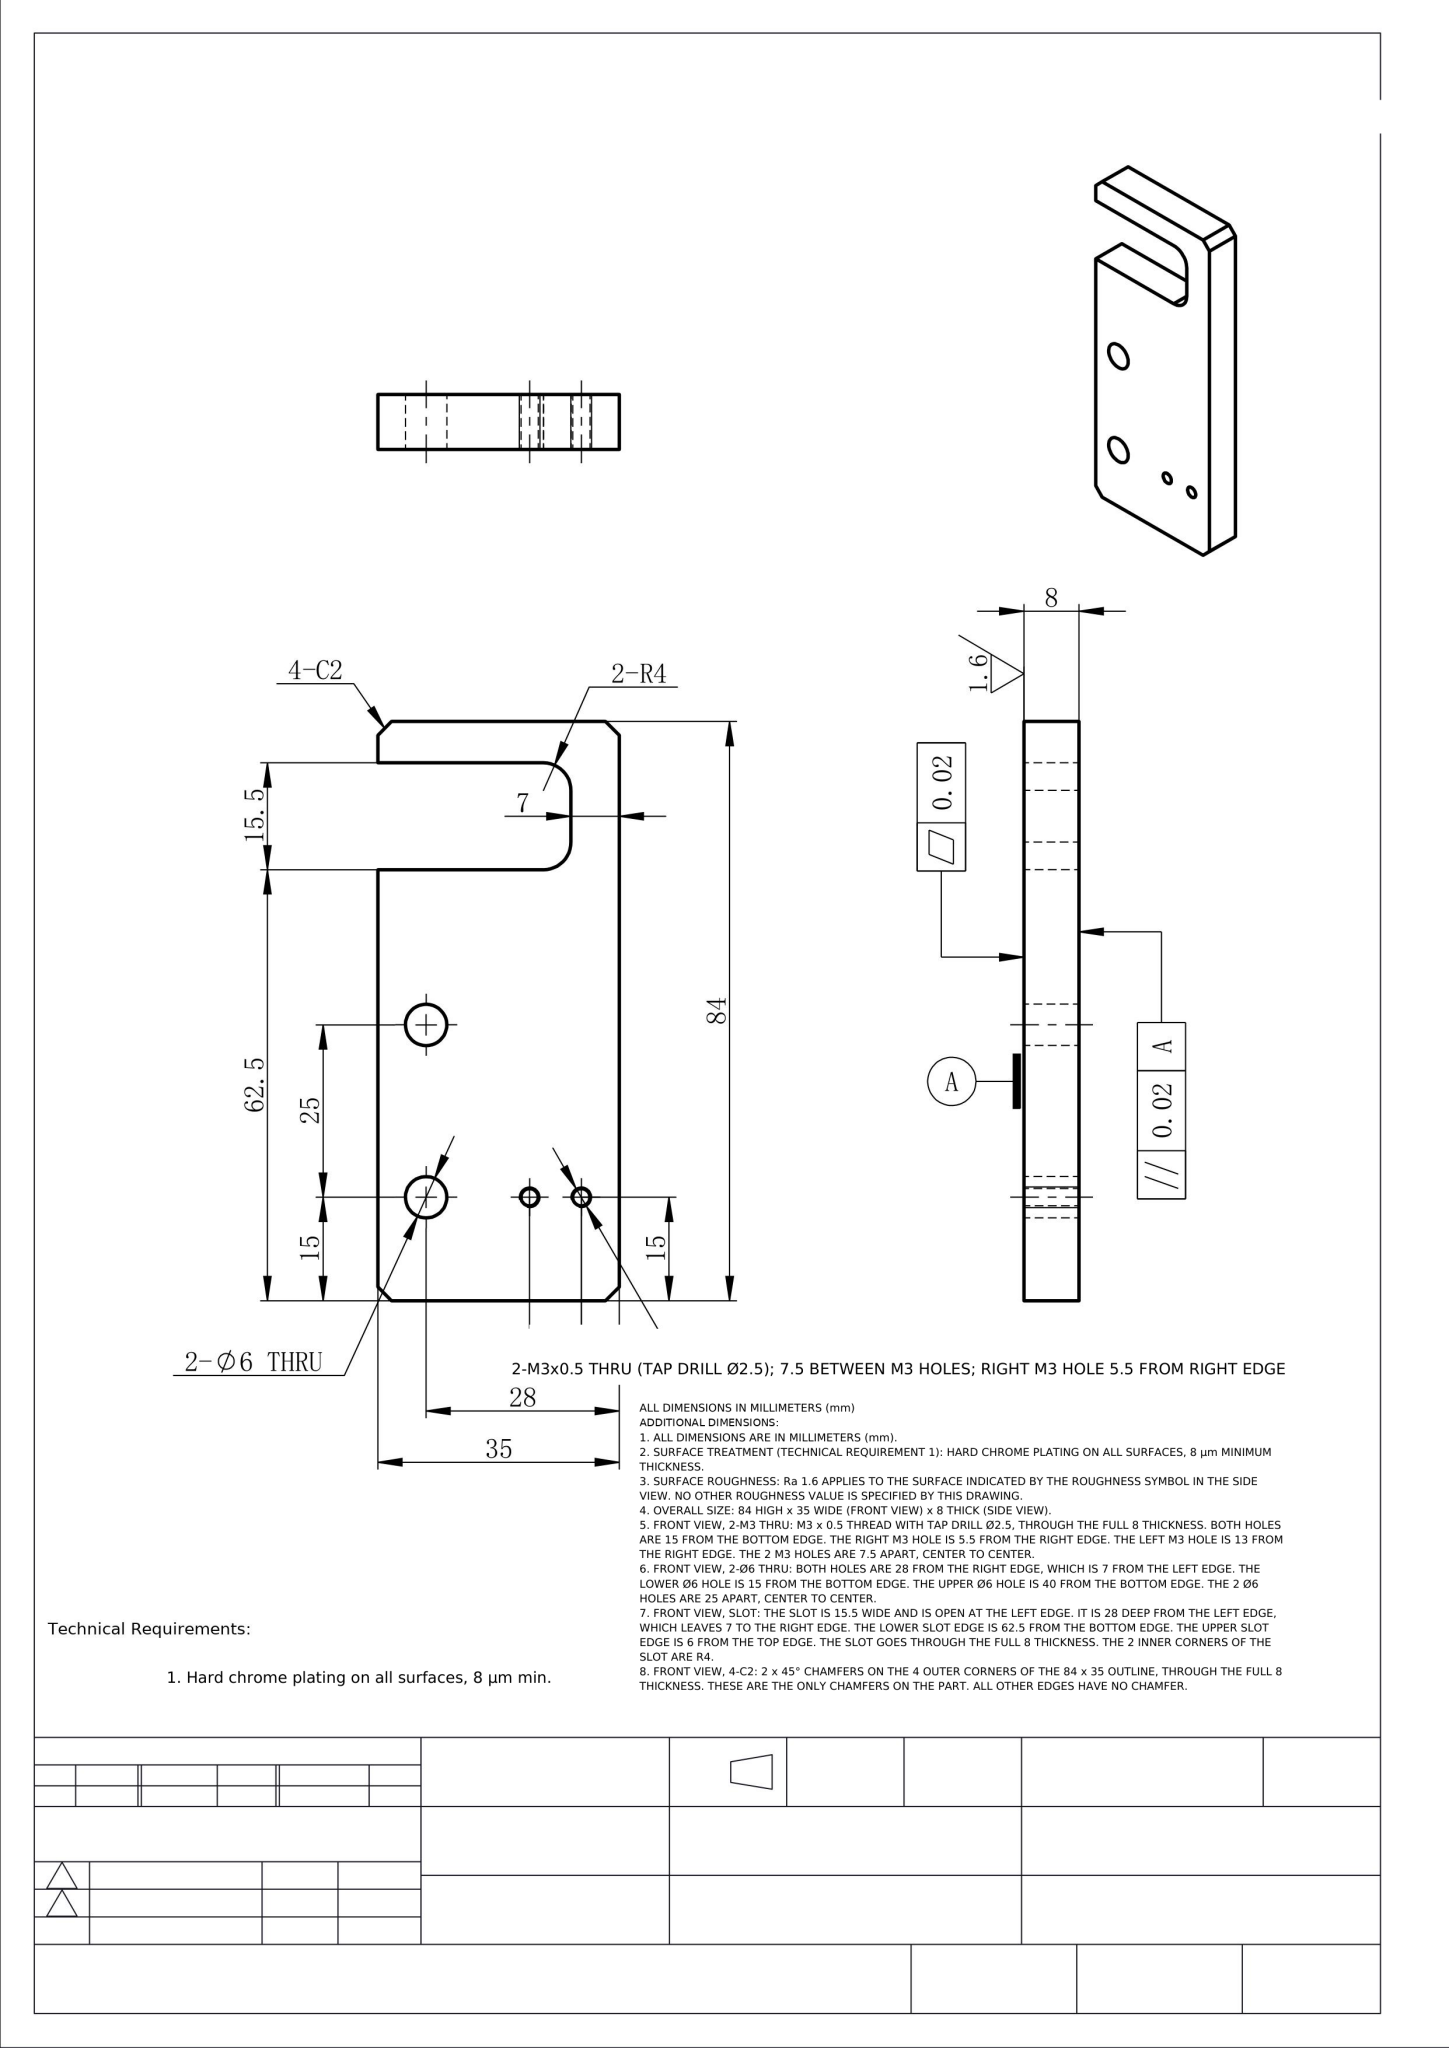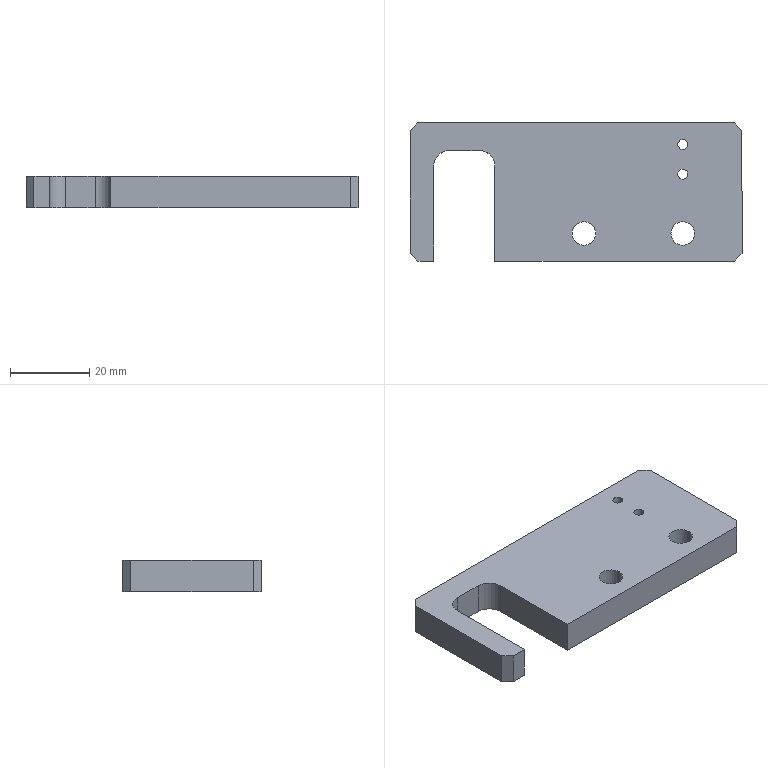Part | NX | mm | 1 solid | 24 faces | box 84 x 35 x 8 mm | volume 19508 mm3 | plane 14 | cylinder 10 | commonest cylinder face diameters 2.5 x4 6 x4 8 x2
STEP:
#1=COLOUR_RGB('',0.7961,0.8235,0.9373);
#2=FILL_AREA_STYLE_COLOUR('',#1);
#3=FILL_AREA_STYLE('',(#2));
#4=SURFACE_STYLE_FILL_AREA(#3);
#5=SURFACE_SIDE_STYLE('',(#4));
#6=SURFACE_STYLE_USAGE(.BOTH.,#5);
#7=PRESENTATION_STYLE_ASSIGNMENT((#6));
#8=CARTESIAN_POINT('',(-16.25,-5.5,-4.));
#9=VERTEX_POINT('',#8);
#10=CARTESIAN_POINT('',(-16.25,-5.5,4.));
#11=VERTEX_POINT('',#10);
#12=CARTESIAN_POINT('',(-16.25,-5.5,4.));
#13=DIRECTION('',(0.,0.,1.));
#14=VECTOR('',#13,1000.);
#15=LINE('',#12,#14);
#16=EDGE_CURVE('',#9,#11,#15,.T.);
#17=ORIENTED_EDGE('',*,*,#16,.F.);
#18=CARTESIAN_POINT('',(-13.75,-5.5,-4.));
#19=VERTEX_POINT('',#18);
#20=CARTESIAN_POINT('',(-15.,-5.5,-4.));
#21=DIRECTION('',(0.,0.,1.));
#22=DIRECTION('',(1.,0.,0.));
#23=AXIS2_PLACEMENT_3D('',#20,#21,#22);
#24=CIRCLE('',#23,1.25);
#25=EDGE_CURVE('',#19,#9,#24,.T.);
#26=ORIENTED_EDGE('',*,*,#25,.F.);
#27=CARTESIAN_POINT('',(-13.75,-5.5,4.));
#28=VERTEX_POINT('',#27);
#29=CARTESIAN_POINT('',(-13.75,-5.5,4.));
#30=DIRECTION('',(0.,0.,1.));
#31=VECTOR('',#30,1000.);
#32=LINE('',#29,#31);
#33=EDGE_CURVE('',#19,#28,#32,.T.);
#34=ORIENTED_EDGE('',*,*,#33,.T.);
#35=CARTESIAN_POINT('',(-15.,-5.5,4.));
#36=DIRECTION('',(0.,0.,1.));
#37=DIRECTION('',(1.,0.,0.));
#38=AXIS2_PLACEMENT_3D('',#35,#36,#37);
#39=CIRCLE('',#38,1.25);
#40=EDGE_CURVE('',#28,#11,#39,.T.);
#41=ORIENTED_EDGE('',*,*,#40,.T.);
#42=EDGE_LOOP('',(#17,#26,#34,#41));
#43=FACE_OUTER_BOUND('',#42,.T.);
#44=CARTESIAN_POINT('',(-15.,-5.5,4.));
#45=DIRECTION('',(0.,0.,1.));
#46=DIRECTION('',(1.,0.,0.));
#47=AXIS2_PLACEMENT_3D('',#44,#45,#46);
#48=CYLINDRICAL_SURFACE('',#47,1.25);
#49=ADVANCED_FACE('',(#43),#48,.F.);
#50=STYLED_ITEM('',(#7),#49);
#51=(LENGTH_UNIT()NAMED_UNIT(*)SI_UNIT(.MILLI.,.METRE.));
#52=UNCERTAINTY_MEASURE_WITH_UNIT(LENGTH_MEASURE(0.00001),#51,'','');
#53=(NAMED_UNIT(*)PLANE_ANGLE_UNIT()SI_UNIT($,.RADIAN.));
#54=(NAMED_UNIT(*)SI_UNIT($,.STERADIAN.)SOLID_ANGLE_UNIT());
#55=(GEOMETRIC_REPRESENTATION_CONTEXT(3)GLOBAL_UNCERTAINTY_ASSIGNED_CONTEXT((#52))GLOBAL_UNIT_ASSIGNED_CONTEXT((#51,#53,#54))REPRESENTATION_CONTEXT('',''));
#56=MECHANICAL_DESIGN_GEOMETRIC_PRESENTATION_REPRESENTATION('',(#50),#55);
#57=COLOUR_RGB('',0.7961,0.8235,0.9373);
#58=FILL_AREA_STYLE_COLOUR('',#57);
#59=FILL_AREA_STYLE('',(#58));
#60=SURFACE_STYLE_FILL_AREA(#59);
#61=SURFACE_SIDE_STYLE('',(#60));
#62=SURFACE_STYLE_USAGE(.BOTH.,#61);
#63=PRESENTATION_STYLE_ASSIGNMENT((#62));
#64=CARTESIAN_POINT('',(-15.,-5.5,-4.));
#65=DIRECTION('',(0.,0.,1.));
#66=DIRECTION('',(1.,0.,0.));
#67=AXIS2_PLACEMENT_3D('',#64,#65,#66);
#68=CIRCLE('',#67,1.25);
#69=EDGE_CURVE('',#9,#19,#68,.T.);
#70=ORIENTED_EDGE('',*,*,#69,.F.);
#71=ORIENTED_EDGE('',*,*,#16,.T.);
#72=CARTESIAN_POINT('',(-15.,-5.5,4.));
#73=DIRECTION('',(0.,0.,1.));
#74=DIRECTION('',(1.,0.,0.));
#75=AXIS2_PLACEMENT_3D('',#72,#73,#74);
#76=CIRCLE('',#75,1.25);
#77=EDGE_CURVE('',#11,#28,#76,.T.);
#78=ORIENTED_EDGE('',*,*,#77,.T.);
#79=ORIENTED_EDGE('',*,*,#33,.F.);
#80=EDGE_LOOP('',(#70,#71,#78,#79));
#81=FACE_OUTER_BOUND('',#80,.T.);
#82=CARTESIAN_POINT('',(-15.,-5.5,4.));
#83=DIRECTION('',(0.,0.,1.));
#84=DIRECTION('',(1.,0.,0.));
#85=AXIS2_PLACEMENT_3D('',#82,#83,#84);
#86=CYLINDRICAL_SURFACE('',#85,1.25);
#87=ADVANCED_FACE('',(#81),#86,.F.);
#88=CARTESIAN_POINT('',(-16.25,-13.,-4.));
#89=VERTEX_POINT('',#88);
#90=CARTESIAN_POINT('',(-13.75,-13.,-4.));
#91=VERTEX_POINT('',#90);
#92=CARTESIAN_POINT('',(-15.,-13.,-4.));
#93=DIRECTION('',(0.,0.,1.));
#94=DIRECTION('',(1.,0.,0.));
#95=AXIS2_PLACEMENT_3D('',#92,#93,#94);
#96=CIRCLE('',#95,1.25);
#97=EDGE_CURVE('',#89,#91,#96,.T.);
#98=ORIENTED_EDGE('',*,*,#97,.F.);
#99=CARTESIAN_POINT('',(-16.25,-13.,4.));
#100=VERTEX_POINT('',#99);
#101=CARTESIAN_POINT('',(-16.25,-13.,4.));
#102=DIRECTION('',(0.,0.,1.));
#103=VECTOR('',#102,1000.);
#104=LINE('',#101,#103);
#105=EDGE_CURVE('',#89,#100,#104,.T.);
#106=ORIENTED_EDGE('',*,*,#105,.T.);
#107=CARTESIAN_POINT('',(-13.75,-13.,4.));
#108=VERTEX_POINT('',#107);
#109=CARTESIAN_POINT('',(-15.,-13.,4.));
#110=DIRECTION('',(0.,0.,1.));
#111=DIRECTION('',(1.,0.,0.));
#112=AXIS2_PLACEMENT_3D('',#109,#110,#111);
#113=CIRCLE('',#112,1.25);
#114=EDGE_CURVE('',#100,#108,#113,.T.);
#115=ORIENTED_EDGE('',*,*,#114,.T.);
#116=CARTESIAN_POINT('',(-13.75,-13.,4.));
#117=DIRECTION('',(0.,0.,1.));
#118=VECTOR('',#117,1000.);
#119=LINE('',#116,#118);
#120=EDGE_CURVE('',#91,#108,#119,.T.);
#121=ORIENTED_EDGE('',*,*,#120,.F.);
#122=EDGE_LOOP('',(#98,#106,#115,#121));
#123=FACE_OUTER_BOUND('',#122,.T.);
#124=CARTESIAN_POINT('',(-15.,-13.,4.));
#125=DIRECTION('',(0.,0.,1.));
#126=DIRECTION('',(1.,0.,0.));
#127=AXIS2_PLACEMENT_3D('',#124,#125,#126);
#128=CYLINDRICAL_SURFACE('',#127,1.25);
#129=ADVANCED_FACE('',(#123),#128,.F.);
#130=CARTESIAN_POINT('',(-18.,-28.,-4.));
#131=VERTEX_POINT('',#130);
#132=CARTESIAN_POINT('',(-12.,-28.,-4.));
#133=VERTEX_POINT('',#132);
#134=CARTESIAN_POINT('',(-15.,-28.,-4.));
#135=DIRECTION('',(0.,0.,1.));
#136=DIRECTION('',(1.,0.,0.));
#137=AXIS2_PLACEMENT_3D('',#134,#135,#136);
#138=CIRCLE('',#137,3.);
#139=EDGE_CURVE('',#131,#133,#138,.T.);
#140=ORIENTED_EDGE('',*,*,#139,.F.);
#141=CARTESIAN_POINT('',(-18.,-28.,4.));
#142=VERTEX_POINT('',#141);
#143=CARTESIAN_POINT('',(-18.,-28.,-4.));
#144=DIRECTION('',(0.,0.,1.));
#145=VECTOR('',#144,1000.);
#146=LINE('',#143,#145);
#147=EDGE_CURVE('',#131,#142,#146,.T.);
#148=ORIENTED_EDGE('',*,*,#147,.T.);
#149=CARTESIAN_POINT('',(-12.,-28.,4.));
#150=VERTEX_POINT('',#149);
#151=CARTESIAN_POINT('',(-15.,-28.,4.));
#152=DIRECTION('',(0.,0.,1.));
#153=DIRECTION('',(1.,0.,0.));
#154=AXIS2_PLACEMENT_3D('',#151,#152,#153);
#155=CIRCLE('',#154,3.);
#156=EDGE_CURVE('',#142,#150,#155,.T.);
#157=ORIENTED_EDGE('',*,*,#156,.T.);
#158=CARTESIAN_POINT('',(-12.,-28.,-4.));
#159=DIRECTION('',(0.,0.,1.));
#160=VECTOR('',#159,1000.);
#161=LINE('',#158,#160);
#162=EDGE_CURVE('',#133,#150,#161,.T.);
#163=ORIENTED_EDGE('',*,*,#162,.F.);
#164=EDGE_LOOP('',(#140,#148,#157,#163));
#165=FACE_OUTER_BOUND('',#164,.T.);
#166=CARTESIAN_POINT('',(-15.,-28.,-4.));
#167=DIRECTION('',(0.,0.,1.));
#168=DIRECTION('',(1.,0.,0.));
#169=AXIS2_PLACEMENT_3D('',#166,#167,#168);
#170=CYLINDRICAL_SURFACE('',#169,3.);
#171=ADVANCED_FACE('',(#165),#170,.F.);
#172=CARTESIAN_POINT('',(-43.,-28.,-4.));
#173=VERTEX_POINT('',#172);
#174=CARTESIAN_POINT('',(-37.,-28.,-4.));
#175=VERTEX_POINT('',#174);
#176=CARTESIAN_POINT('',(-40.,-28.,-4.));
#177=DIRECTION('',(0.,0.,1.));
#178=DIRECTION('',(1.,0.,0.));
#179=AXIS2_PLACEMENT_3D('',#176,#177,#178);
#180=CIRCLE('',#179,3.);
#181=EDGE_CURVE('',#173,#175,#180,.T.);
#182=ORIENTED_EDGE('',*,*,#181,.F.);
#183=CARTESIAN_POINT('',(-43.,-28.,4.));
#184=VERTEX_POINT('',#183);
#185=CARTESIAN_POINT('',(-43.,-28.,-4.));
#186=DIRECTION('',(0.,0.,1.));
#187=VECTOR('',#186,1000.);
#188=LINE('',#185,#187);
#189=EDGE_CURVE('',#173,#184,#188,.T.);
#190=ORIENTED_EDGE('',*,*,#189,.T.);
#191=CARTESIAN_POINT('',(-37.,-28.,4.));
#192=VERTEX_POINT('',#191);
#193=CARTESIAN_POINT('',(-40.,-28.,4.));
#194=DIRECTION('',(0.,0.,1.));
#195=DIRECTION('',(1.,0.,0.));
#196=AXIS2_PLACEMENT_3D('',#193,#194,#195);
#197=CIRCLE('',#196,3.);
#198=EDGE_CURVE('',#184,#192,#197,.T.);
#199=ORIENTED_EDGE('',*,*,#198,.T.);
#200=CARTESIAN_POINT('',(-37.,-28.,-4.));
#201=DIRECTION('',(0.,0.,1.));
#202=VECTOR('',#201,1000.);
#203=LINE('',#200,#202);
#204=EDGE_CURVE('',#175,#192,#203,.T.);
#205=ORIENTED_EDGE('',*,*,#204,.F.);
#206=EDGE_LOOP('',(#182,#190,#199,#205));
#207=FACE_OUTER_BOUND('',#206,.T.);
#208=CARTESIAN_POINT('',(-40.,-28.,-4.));
#209=DIRECTION('',(0.,0.,1.));
#210=DIRECTION('',(1.,0.,0.));
#211=AXIS2_PLACEMENT_3D('',#208,#209,#210);
#212=CYLINDRICAL_SURFACE('',#211,3.);
#213=ADVANCED_FACE('',(#207),#212,.F.);
#214=CARTESIAN_POINT('',(0.,-33.,4.));
#215=VERTEX_POINT('',#214);
#216=CARTESIAN_POINT('',(0.,-2.,4.));
#217=VERTEX_POINT('',#216);
#218=CARTESIAN_POINT('',(0.,0.,4.));
#219=DIRECTION('',(-0.,1.,0.));
#220=VECTOR('',#219,1000.);
#221=LINE('',#218,#220);
#222=EDGE_CURVE('',#215,#217,#221,.T.);
#223=ORIENTED_EDGE('',*,*,#222,.F.);
#224=CARTESIAN_POINT('',(0.,-33.,-4.));
#225=VERTEX_POINT('',#224);
#226=CARTESIAN_POINT('',(0.,-33.,4.));
#227=DIRECTION('',(0.,0.,-1.));
#228=VECTOR('',#227,1000.);
#229=LINE('',#226,#228);
#230=EDGE_CURVE('',#215,#225,#229,.T.);
#231=ORIENTED_EDGE('',*,*,#230,.T.);
#232=CARTESIAN_POINT('',(0.,-2.,-4.));
#233=VERTEX_POINT('',#232);
#234=CARTESIAN_POINT('',(0.,0.,-4.));
#235=DIRECTION('',(-0.,1.,0.));
#236=VECTOR('',#235,1000.);
#237=LINE('',#234,#236);
#238=EDGE_CURVE('',#225,#233,#237,.T.);
#239=ORIENTED_EDGE('',*,*,#238,.T.);
#240=CARTESIAN_POINT('',(0.,-2.,4.));
#241=DIRECTION('',(0.,0.,1.));
#242=VECTOR('',#241,1000.);
#243=LINE('',#240,#242);
#244=EDGE_CURVE('',#233,#217,#243,.T.);
#245=ORIENTED_EDGE('',*,*,#244,.T.);
#246=EDGE_LOOP('',(#223,#231,#239,#245));
#247=FACE_OUTER_BOUND('',#246,.T.);
#248=CARTESIAN_POINT('',(0.,0.,4.));
#249=DIRECTION('',(-1.,-0.,0.));
#250=DIRECTION('',(0.,-1.,0.));
#251=AXIS2_PLACEMENT_3D('',#248,#249,#250);
#252=PLANE('',#251);
#253=ADVANCED_FACE('',(#247),#252,.F.);
#254=CARTESIAN_POINT('',(-2.,-0.,4.));
#255=VERTEX_POINT('',#254);
#256=CARTESIAN_POINT('',(-82.,-0.,4.));
#257=VERTEX_POINT('',#256);
#258=CARTESIAN_POINT('',(0.,0.,4.));
#259=DIRECTION('',(-1.,-0.,0.));
#260=VECTOR('',#259,1000.);
#261=LINE('',#258,#260);
#262=EDGE_CURVE('',#255,#257,#261,.T.);
#263=ORIENTED_EDGE('',*,*,#262,.F.);
#264=CARTESIAN_POINT('',(-2.,0.,-4.));
#265=VERTEX_POINT('',#264);
#266=CARTESIAN_POINT('',(-2.,-0.,4.));
#267=DIRECTION('',(0.,0.,-1.));
#268=VECTOR('',#267,1000.);
#269=LINE('',#266,#268);
#270=EDGE_CURVE('',#255,#265,#269,.T.);
#271=ORIENTED_EDGE('',*,*,#270,.T.);
#272=CARTESIAN_POINT('',(-82.,-0.,-4.));
#273=VERTEX_POINT('',#272);
#274=CARTESIAN_POINT('',(0.,0.,-4.));
#275=DIRECTION('',(-1.,-0.,0.));
#276=VECTOR('',#275,1000.);
#277=LINE('',#274,#276);
#278=EDGE_CURVE('',#265,#273,#277,.T.);
#279=ORIENTED_EDGE('',*,*,#278,.T.);
#280=CARTESIAN_POINT('',(-82.,-0.,4.));
#281=DIRECTION('',(0.,0.,1.));
#282=VECTOR('',#281,1000.);
#283=LINE('',#280,#282);
#284=EDGE_CURVE('',#273,#257,#283,.T.);
#285=ORIENTED_EDGE('',*,*,#284,.T.);
#286=EDGE_LOOP('',(#263,#271,#279,#285));
#287=FACE_OUTER_BOUND('',#286,.T.);
#288=CARTESIAN_POINT('',(0.,0.,4.));
#289=DIRECTION('',(0.,-1.,0.));
#290=DIRECTION('',(1.,0.,0.));
#291=AXIS2_PLACEMENT_3D('',#288,#289,#290);
#292=PLANE('',#291);
#293=ADVANCED_FACE('',(#287),#292,.F.);
#294=CARTESIAN_POINT('',(-84.,-2.,-4.));
#295=VERTEX_POINT('',#294);
#296=CARTESIAN_POINT('',(-84.,-33.,-4.));
#297=VERTEX_POINT('',#296);
#298=CARTESIAN_POINT('',(-84.,-35.,-4.));
#299=DIRECTION('',(0.,-1.,0.));
#300=VECTOR('',#299,1000.);
#301=LINE('',#298,#300);
#302=EDGE_CURVE('',#295,#297,#301,.T.);
#303=ORIENTED_EDGE('',*,*,#302,.T.);
#304=CARTESIAN_POINT('',(-84.,-33.,4.));
#305=VERTEX_POINT('',#304);
#306=CARTESIAN_POINT('',(-84.,-33.,4.));
#307=DIRECTION('',(0.,0.,1.));
#308=VECTOR('',#307,1000.);
#309=LINE('',#306,#308);
#310=EDGE_CURVE('',#297,#305,#309,.T.);
#311=ORIENTED_EDGE('',*,*,#310,.T.);
#312=CARTESIAN_POINT('',(-84.,-2.,4.));
#313=VERTEX_POINT('',#312);
#314=CARTESIAN_POINT('',(-84.,-35.,4.));
#315=DIRECTION('',(0.,-1.,0.));
#316=VECTOR('',#315,1000.);
#317=LINE('',#314,#316);
#318=EDGE_CURVE('',#313,#305,#317,.T.);
#319=ORIENTED_EDGE('',*,*,#318,.F.);
#320=CARTESIAN_POINT('',(-84.,-2.,4.));
#321=DIRECTION('',(0.,0.,-1.));
#322=VECTOR('',#321,1000.);
#323=LINE('',#320,#322);
#324=EDGE_CURVE('',#313,#295,#323,.T.);
#325=ORIENTED_EDGE('',*,*,#324,.T.);
#326=EDGE_LOOP('',(#303,#311,#319,#325));
#327=FACE_OUTER_BOUND('',#326,.T.);
#328=CARTESIAN_POINT('',(-84.,-35.,4.));
#329=DIRECTION('',(1.,0.,0.));
#330=DIRECTION('',(0.,0.,-1.));
#331=AXIS2_PLACEMENT_3D('',#328,#329,#330);
#332=PLANE('',#331);
#333=ADVANCED_FACE('',(#327),#332,.F.);
#334=CARTESIAN_POINT('',(-82.,-35.,4.));
#335=VERTEX_POINT('',#334);
#336=CARTESIAN_POINT('',(-78.,-35.,4.));
#337=VERTEX_POINT('',#336);
#338=CARTESIAN_POINT('',(-78.,-35.,4.));
#339=DIRECTION('',(1.,-0.,0.));
#340=VECTOR('',#339,1000.);
#341=LINE('',#338,#340);
#342=EDGE_CURVE('',#335,#337,#341,.T.);
#343=ORIENTED_EDGE('',*,*,#342,.F.);
#344=CARTESIAN_POINT('',(-82.,-35.,-4.));
#345=VERTEX_POINT('',#344);
#346=CARTESIAN_POINT('',(-82.,-35.,4.));
#347=DIRECTION('',(0.,0.,-1.));
#348=VECTOR('',#347,1000.);
#349=LINE('',#346,#348);
#350=EDGE_CURVE('',#335,#345,#349,.T.);
#351=ORIENTED_EDGE('',*,*,#350,.T.);
#352=CARTESIAN_POINT('',(-78.,-35.,-4.));
#353=VERTEX_POINT('',#352);
#354=CARTESIAN_POINT('',(-78.,-35.,-4.));
#355=DIRECTION('',(1.,-0.,0.));
#356=VECTOR('',#355,1000.);
#357=LINE('',#354,#356);
#358=EDGE_CURVE('',#345,#353,#357,.T.);
#359=ORIENTED_EDGE('',*,*,#358,.T.);
#360=CARTESIAN_POINT('',(-78.,-35.,4.));
#361=DIRECTION('',(0.,0.,-1.));
#362=VECTOR('',#361,1000.);
#363=LINE('',#360,#362);
#364=EDGE_CURVE('',#337,#353,#363,.T.);
#365=ORIENTED_EDGE('',*,*,#364,.F.);
#366=EDGE_LOOP('',(#343,#351,#359,#365));
#367=FACE_OUTER_BOUND('',#366,.T.);
#368=CARTESIAN_POINT('',(-78.,-35.,4.));
#369=DIRECTION('',(0.,1.,0.));
#370=DIRECTION('',(-1.,0.,0.));
#371=AXIS2_PLACEMENT_3D('',#368,#369,#370);
#372=PLANE('',#371);
#373=ADVANCED_FACE('',(#367),#372,.F.);
#374=CARTESIAN_POINT('',(-78.,-11.,-4.));
#375=VERTEX_POINT('',#374);
#376=CARTESIAN_POINT('',(-78.,-7.,-4.));
#377=DIRECTION('',(0.,1.,0.));
#378=VECTOR('',#377,1000.);
#379=LINE('',#376,#378);
#380=EDGE_CURVE('',#353,#375,#379,.T.);
#381=ORIENTED_EDGE('',*,*,#380,.T.);
#382=CARTESIAN_POINT('',(-78.,-11.,4.));
#383=VERTEX_POINT('',#382);
#384=CARTESIAN_POINT('',(-78.,-11.,4.));
#385=DIRECTION('',(0.,0.,1.));
#386=VECTOR('',#385,1000.);
#387=LINE('',#384,#386);
#388=EDGE_CURVE('',#375,#383,#387,.T.);
#389=ORIENTED_EDGE('',*,*,#388,.T.);
#390=CARTESIAN_POINT('',(-78.,-7.,4.));
#391=DIRECTION('',(0.,1.,0.));
#392=VECTOR('',#391,1000.);
#393=LINE('',#390,#392);
#394=EDGE_CURVE('',#337,#383,#393,.T.);
#395=ORIENTED_EDGE('',*,*,#394,.F.);
#396=ORIENTED_EDGE('',*,*,#364,.T.);
#397=EDGE_LOOP('',(#381,#389,#395,#396));
#398=FACE_OUTER_BOUND('',#397,.T.);
#399=CARTESIAN_POINT('',(-78.,-7.,4.));
#400=DIRECTION('',(-1.,0.,0.));
#401=DIRECTION('',(0.,0.,1.));
#402=AXIS2_PLACEMENT_3D('',#399,#400,#401);
#403=PLANE('',#402);
#404=ADVANCED_FACE('',(#398),#403,.F.);
#405=CARTESIAN_POINT('',(-74.,-7.,-4.));
#406=VERTEX_POINT('',#405);
#407=CARTESIAN_POINT('',(-66.5,-7.,-4.));
#408=VERTEX_POINT('',#407);
#409=CARTESIAN_POINT('',(-62.5,-7.,-4.));
#410=DIRECTION('',(1.,0.,0.));
#411=VECTOR('',#410,1000.);
#412=LINE('',#409,#411);
#413=EDGE_CURVE('',#406,#408,#412,.T.);
#414=ORIENTED_EDGE('',*,*,#413,.T.);
#415=CARTESIAN_POINT('',(-66.5,-7.,4.));
#416=VERTEX_POINT('',#415);
#417=CARTESIAN_POINT('',(-66.5,-7.,4.));
#418=DIRECTION('',(0.,0.,1.));
#419=VECTOR('',#418,1000.);
#420=LINE('',#417,#419);
#421=EDGE_CURVE('',#408,#416,#420,.T.);
#422=ORIENTED_EDGE('',*,*,#421,.T.);
#423=CARTESIAN_POINT('',(-74.,-7.,4.));
#424=VERTEX_POINT('',#423);
#425=CARTESIAN_POINT('',(-62.5,-7.,4.));
#426=DIRECTION('',(1.,0.,0.));
#427=VECTOR('',#426,1000.);
#428=LINE('',#425,#427);
#429=EDGE_CURVE('',#424,#416,#428,.T.);
#430=ORIENTED_EDGE('',*,*,#429,.F.);
#431=CARTESIAN_POINT('',(-74.,-7.,-4.));
#432=DIRECTION('',(0.,0.,-1.));
#433=VECTOR('',#432,1000.);
#434=LINE('',#431,#433);
#435=EDGE_CURVE('',#424,#406,#434,.T.);
#436=ORIENTED_EDGE('',*,*,#435,.T.);
#437=EDGE_LOOP('',(#414,#422,#430,#436));
#438=FACE_OUTER_BOUND('',#437,.T.);
#439=CARTESIAN_POINT('',(-62.5,-7.,4.));
#440=DIRECTION('',(-0.,1.,0.));
#441=DIRECTION('',(-1.,-0.,0.));
#442=AXIS2_PLACEMENT_3D('',#439,#440,#441);
#443=PLANE('',#442);
#444=ADVANCED_FACE('',(#438),#443,.F.);
#445=CARTESIAN_POINT('',(-62.5,-11.,4.));
#446=VERTEX_POINT('',#445);
#447=CARTESIAN_POINT('',(-62.5,-35.,4.));
#448=VERTEX_POINT('',#447);
#449=CARTESIAN_POINT('',(-62.5,-35.,4.));
#450=DIRECTION('',(0.,-1.,0.));
#451=VECTOR('',#450,1000.);
#452=LINE('',#449,#451);
#453=EDGE_CURVE('',#446,#448,#452,.T.);
#454=ORIENTED_EDGE('',*,*,#453,.F.);
#455=CARTESIAN_POINT('',(-62.5,-11.,-4.));
#456=VERTEX_POINT('',#455);
#457=CARTESIAN_POINT('',(-62.5,-11.,-4.));
#458=DIRECTION('',(0.,0.,-1.));
#459=VECTOR('',#458,1000.);
#460=LINE('',#457,#459);
#461=EDGE_CURVE('',#446,#456,#460,.T.);
#462=ORIENTED_EDGE('',*,*,#461,.T.);
#463=CARTESIAN_POINT('',(-62.5,-35.,-4.));
#464=VERTEX_POINT('',#463);
#465=CARTESIAN_POINT('',(-62.5,-35.,-4.));
#466=DIRECTION('',(0.,-1.,0.));
#467=VECTOR('',#466,1000.);
#468=LINE('',#465,#467);
#469=EDGE_CURVE('',#456,#464,#468,.T.);
#470=ORIENTED_EDGE('',*,*,#469,.T.);
#471=CARTESIAN_POINT('',(-62.5,-35.,4.));
#472=DIRECTION('',(0.,0.,-1.));
#473=VECTOR('',#472,1000.);
#474=LINE('',#471,#473);
#475=EDGE_CURVE('',#448,#464,#474,.T.);
#476=ORIENTED_EDGE('',*,*,#475,.F.);
#477=EDGE_LOOP('',(#454,#462,#470,#476));
#478=FACE_OUTER_BOUND('',#477,.T.);
#479=CARTESIAN_POINT('',(-62.5,-35.,4.));
#480=DIRECTION('',(1.,0.,0.));
#481=DIRECTION('',(0.,0.,-1.));
#482=AXIS2_PLACEMENT_3D('',#479,#480,#481);
#483=PLANE('',#482);
#484=ADVANCED_FACE('',(#478),#483,.F.);
#485=CARTESIAN_POINT('',(-2.,-35.,-4.));
#486=VERTEX_POINT('',#485);
#487=CARTESIAN_POINT('',(0.,-35.,-4.));
#488=DIRECTION('',(1.,0.,0.));
#489=VECTOR('',#488,1000.);
#490=LINE('',#487,#489);
#491=EDGE_CURVE('',#464,#486,#490,.T.);
#492=ORIENTED_EDGE('',*,*,#491,.T.);
#493=CARTESIAN_POINT('',(-2.,-35.,4.));
#494=VERTEX_POINT('',#493);
#495=CARTESIAN_POINT('',(-2.,-35.,4.));
#496=DIRECTION('',(0.,0.,1.));
#497=VECTOR('',#496,1000.);
#498=LINE('',#495,#497);
#499=EDGE_CURVE('',#486,#494,#498,.T.);
#500=ORIENTED_EDGE('',*,*,#499,.T.);
#501=CARTESIAN_POINT('',(0.,-35.,4.));
#502=DIRECTION('',(1.,0.,0.));
#503=VECTOR('',#502,1000.);
#504=LINE('',#501,#503);
#505=EDGE_CURVE('',#448,#494,#504,.T.);
#506=ORIENTED_EDGE('',*,*,#505,.F.);
#507=ORIENTED_EDGE('',*,*,#475,.T.);
#508=EDGE_LOOP('',(#492,#500,#506,#507));
#509=FACE_OUTER_BOUND('',#508,.T.);
#510=CARTESIAN_POINT('',(0.,-35.,4.));
#511=DIRECTION('',(-0.,1.,0.));
#512=DIRECTION('',(-1.,-0.,0.));
#513=AXIS2_PLACEMENT_3D('',#510,#511,#512);
#514=PLANE('',#513);
#515=ADVANCED_FACE('',(#509),#514,.F.);
#516=ORIENTED_EDGE('',*,*,#40,.F.);
#517=ORIENTED_EDGE('',*,*,#77,.F.);
#518=EDGE_LOOP('',(#516,#517));
#519=FACE_BOUND('',#518,.T.);
#520=CARTESIAN_POINT('',(-15.,-13.,4.));
#521=DIRECTION('',(0.,0.,1.));
#522=DIRECTION('',(1.,0.,0.));
#523=AXIS2_PLACEMENT_3D('',#520,#521,#522);
#524=CIRCLE('',#523,1.25);
#525=EDGE_CURVE('',#108,#100,#524,.T.);
#526=ORIENTED_EDGE('',*,*,#525,.F.);
#527=ORIENTED_EDGE('',*,*,#114,.F.);
#528=EDGE_LOOP('',(#526,#527));
#529=FACE_BOUND('',#528,.T.);
#530=CARTESIAN_POINT('',(-15.,-28.,4.));
#531=DIRECTION('',(0.,0.,1.));
#532=DIRECTION('',(1.,0.,0.));
#533=AXIS2_PLACEMENT_3D('',#530,#531,#532);
#534=CIRCLE('',#533,3.);
#535=EDGE_CURVE('',#150,#142,#534,.T.);
#536=ORIENTED_EDGE('',*,*,#535,.F.);
#537=ORIENTED_EDGE('',*,*,#156,.F.);
#538=EDGE_LOOP('',(#536,#537));
#539=FACE_BOUND('',#538,.T.);
#540=CARTESIAN_POINT('',(-40.,-28.,4.));
#541=DIRECTION('',(0.,0.,1.));
#542=DIRECTION('',(1.,0.,0.));
#543=AXIS2_PLACEMENT_3D('',#540,#541,#542);
#544=CIRCLE('',#543,3.);
#545=EDGE_CURVE('',#192,#184,#544,.T.);
#546=ORIENTED_EDGE('',*,*,#545,.F.);
#547=ORIENTED_EDGE('',*,*,#198,.F.);
#548=EDGE_LOOP('',(#546,#547));
#549=FACE_BOUND('',#548,.T.);
#550=ORIENTED_EDGE('',*,*,#318,.T.);
#551=CARTESIAN_POINT('',(-82.,-35.,4.));
#552=DIRECTION('',(0.7071,-0.7071,0.));
#553=VECTOR('',#552,1000.);
#554=LINE('',#551,#553);
#555=EDGE_CURVE('',#305,#335,#554,.T.);
#556=ORIENTED_EDGE('',*,*,#555,.T.);
#557=ORIENTED_EDGE('',*,*,#342,.T.);
#558=ORIENTED_EDGE('',*,*,#394,.T.);
#559=CARTESIAN_POINT('',(-74.,-11.,4.));
#560=DIRECTION('',(0.,0.,-1.));
#561=DIRECTION('',(-1.,0.,0.));
#562=AXIS2_PLACEMENT_3D('',#559,#560,#561);
#563=CIRCLE('',#562,4.);
#564=EDGE_CURVE('',#383,#424,#563,.T.);
#565=ORIENTED_EDGE('',*,*,#564,.T.);
#566=ORIENTED_EDGE('',*,*,#429,.T.);
#567=CARTESIAN_POINT('',(-66.5,-11.,4.));
#568=DIRECTION('',(0.,0.,-1.));
#569=DIRECTION('',(-1.,0.,0.));
#570=AXIS2_PLACEMENT_3D('',#567,#568,#569);
#571=CIRCLE('',#570,4.);
#572=EDGE_CURVE('',#416,#446,#571,.T.);
#573=ORIENTED_EDGE('',*,*,#572,.T.);
#574=ORIENTED_EDGE('',*,*,#453,.T.);
#575=ORIENTED_EDGE('',*,*,#505,.T.);
#576=CARTESIAN_POINT('',(0.,-33.,4.));
#577=DIRECTION('',(0.7071,0.7071,0.));
#578=VECTOR('',#577,1000.);
#579=LINE('',#576,#578);
#580=EDGE_CURVE('',#494,#215,#579,.T.);
#581=ORIENTED_EDGE('',*,*,#580,.T.);
#582=ORIENTED_EDGE('',*,*,#222,.T.);
#583=CARTESIAN_POINT('',(-2.,-0.,4.));
#584=DIRECTION('',(-0.7071,0.7071,0.));
#585=VECTOR('',#584,1000.);
#586=LINE('',#583,#585);
#587=EDGE_CURVE('',#217,#255,#586,.T.);
#588=ORIENTED_EDGE('',*,*,#587,.T.);
#589=ORIENTED_EDGE('',*,*,#262,.T.);
#590=CARTESIAN_POINT('',(-84.,-2.,4.));
#591=DIRECTION('',(-0.7071,-0.7071,0.));
#592=VECTOR('',#591,1000.);
#593=LINE('',#590,#592);
#594=EDGE_CURVE('',#257,#313,#593,.T.);
#595=ORIENTED_EDGE('',*,*,#594,.T.);
#596=EDGE_LOOP('',(#550,#556,#557,#558,#565,#566,#573,#574,#575,#581,#582,#588,#589,#595));
#597=FACE_OUTER_BOUND('',#596,.T.);
#598=CARTESIAN_POINT('',(0.,-35.,4.));
#599=DIRECTION('',(0.,0.,-1.));
#600=DIRECTION('',(-1.,0.,0.));
#601=AXIS2_PLACEMENT_3D('',#598,#599,#600);
#602=PLANE('',#601);
#603=ADVANCED_FACE('',(#519,#529,#539,#549,#597),#602,.F.);
#604=ORIENTED_EDGE('',*,*,#25,.T.);
#605=ORIENTED_EDGE('',*,*,#69,.T.);
#606=EDGE_LOOP('',(#604,#605));
#607=FACE_BOUND('',#606,.T.);
#608=CARTESIAN_POINT('',(-15.,-13.,-4.));
#609=DIRECTION('',(0.,0.,1.));
#610=DIRECTION('',(1.,0.,0.));
#611=AXIS2_PLACEMENT_3D('',#608,#609,#610);
#612=CIRCLE('',#611,1.25);
#613=EDGE_CURVE('',#91,#89,#612,.T.);
#614=ORIENTED_EDGE('',*,*,#613,.T.);
#615=ORIENTED_EDGE('',*,*,#97,.T.);
#616=EDGE_LOOP('',(#614,#615));
#617=FACE_BOUND('',#616,.T.);
#618=CARTESIAN_POINT('',(-15.,-28.,-4.));
#619=DIRECTION('',(0.,0.,1.));
#620=DIRECTION('',(1.,0.,0.));
#621=AXIS2_PLACEMENT_3D('',#618,#619,#620);
#622=CIRCLE('',#621,3.);
#623=EDGE_CURVE('',#133,#131,#622,.T.);
#624=ORIENTED_EDGE('',*,*,#623,.T.);
#625=ORIENTED_EDGE('',*,*,#139,.T.);
#626=EDGE_LOOP('',(#624,#625));
#627=FACE_BOUND('',#626,.T.);
#628=CARTESIAN_POINT('',(-40.,-28.,-4.));
#629=DIRECTION('',(0.,0.,1.));
#630=DIRECTION('',(1.,0.,0.));
#631=AXIS2_PLACEMENT_3D('',#628,#629,#630);
#632=CIRCLE('',#631,3.);
#633=EDGE_CURVE('',#175,#173,#632,.T.);
#634=ORIENTED_EDGE('',*,*,#633,.T.);
#635=ORIENTED_EDGE('',*,*,#181,.T.);
#636=EDGE_LOOP('',(#634,#635));
#637=FACE_BOUND('',#636,.T.);
#638=ORIENTED_EDGE('',*,*,#358,.F.);
#639=CARTESIAN_POINT('',(-41.,-76.,-4.));
#640=DIRECTION('',(-0.7071,0.7071,0.));
#641=VECTOR('',#640,1000.);
#642=LINE('',#639,#641);
#643=EDGE_CURVE('',#345,#297,#642,.T.);
#644=ORIENTED_EDGE('',*,*,#643,.T.);
#645=ORIENTED_EDGE('',*,*,#302,.F.);
#646=CARTESIAN_POINT('',(-58.5,23.5,-4.));
#647=DIRECTION('',(0.7071,0.7071,0.));
#648=VECTOR('',#647,1000.);
#649=LINE('',#646,#648);
#650=EDGE_CURVE('',#295,#273,#649,.T.);
#651=ORIENTED_EDGE('',*,*,#650,.T.);
#652=ORIENTED_EDGE('',*,*,#278,.F.);
#653=CARTESIAN_POINT('',(16.5,-18.5,-4.));
#654=DIRECTION('',(0.7071,-0.7071,0.));
#655=VECTOR('',#654,1000.);
#656=LINE('',#653,#655);
#657=EDGE_CURVE('',#265,#233,#656,.T.);
#658=ORIENTED_EDGE('',*,*,#657,.T.);
#659=ORIENTED_EDGE('',*,*,#238,.F.);
#660=CARTESIAN_POINT('',(-1.,-34.,-4.));
#661=DIRECTION('',(-0.7071,-0.7071,0.));
#662=VECTOR('',#661,1000.);
#663=LINE('',#660,#662);
#664=EDGE_CURVE('',#225,#486,#663,.T.);
#665=ORIENTED_EDGE('',*,*,#664,.T.);
#666=ORIENTED_EDGE('',*,*,#491,.F.);
#667=ORIENTED_EDGE('',*,*,#469,.F.);
#668=CARTESIAN_POINT('',(-66.5,-11.,-4.));
#669=DIRECTION('',(0.,0.,1.));
#670=DIRECTION('',(-1.,0.,0.));
#671=AXIS2_PLACEMENT_3D('',#668,#669,#670);
#672=CIRCLE('',#671,4.);
#673=EDGE_CURVE('',#456,#408,#672,.T.);
#674=ORIENTED_EDGE('',*,*,#673,.T.);
#675=ORIENTED_EDGE('',*,*,#413,.F.);
#676=CARTESIAN_POINT('',(-74.,-11.,-4.));
#677=DIRECTION('',(0.,0.,1.));
#678=DIRECTION('',(-1.,0.,0.));
#679=AXIS2_PLACEMENT_3D('',#676,#677,#678);
#680=CIRCLE('',#679,4.);
#681=EDGE_CURVE('',#406,#375,#680,.T.);
#682=ORIENTED_EDGE('',*,*,#681,.T.);
#683=ORIENTED_EDGE('',*,*,#380,.F.);
#684=EDGE_LOOP('',(#638,#644,#645,#651,#652,#658,#659,#665,#666,#667,#674,#675,#682,#683));
#685=FACE_OUTER_BOUND('',#684,.T.);
#686=CARTESIAN_POINT('',(0.,-35.,-4.));
#687=DIRECTION('',(0.,0.,-1.));
#688=DIRECTION('',(-1.,0.,0.));
#689=AXIS2_PLACEMENT_3D('',#686,#687,#688);
#690=PLANE('',#689);
#691=ADVANCED_FACE('',(#607,#617,#627,#637,#685),#690,.T.);
#692=ORIENTED_EDGE('',*,*,#572,.F.);
#693=ORIENTED_EDGE('',*,*,#421,.F.);
#694=ORIENTED_EDGE('',*,*,#673,.F.);
#695=ORIENTED_EDGE('',*,*,#461,.F.);
#696=EDGE_LOOP('',(#692,#693,#694,#695));
#697=FACE_OUTER_BOUND('',#696,.T.);
#698=CARTESIAN_POINT('',(-66.5,-11.,4.));
#699=DIRECTION('',(0.,0.,1.));
#700=DIRECTION('',(1.,0.,0.));
#701=AXIS2_PLACEMENT_3D('',#698,#699,#700);
#702=CYLINDRICAL_SURFACE('',#701,4.);
#703=ADVANCED_FACE('',(#697),#702,.F.);
#704=ORIENTED_EDGE('',*,*,#564,.F.);
#705=ORIENTED_EDGE('',*,*,#388,.F.);
#706=ORIENTED_EDGE('',*,*,#681,.F.);
#707=ORIENTED_EDGE('',*,*,#435,.F.);
#708=EDGE_LOOP('',(#704,#705,#706,#707));
#709=FACE_OUTER_BOUND('',#708,.T.);
#710=CARTESIAN_POINT('',(-74.,-11.,4.));
#711=DIRECTION('',(0.,0.,1.));
#712=DIRECTION('',(1.,0.,0.));
#713=AXIS2_PLACEMENT_3D('',#710,#711,#712);
#714=CYLINDRICAL_SURFACE('',#713,4.);
#715=ADVANCED_FACE('',(#709),#714,.F.);
#716=ORIENTED_EDGE('',*,*,#189,.F.);
#717=ORIENTED_EDGE('',*,*,#633,.F.);
#718=ORIENTED_EDGE('',*,*,#204,.T.);
#719=ORIENTED_EDGE('',*,*,#545,.T.);
#720=EDGE_LOOP('',(#716,#717,#718,#719));
#721=FACE_OUTER_BOUND('',#720,.T.);
#722=CARTESIAN_POINT('',(-40.,-28.,-4.));
#723=DIRECTION('',(0.,0.,1.));
#724=DIRECTION('',(1.,0.,0.));
#725=AXIS2_PLACEMENT_3D('',#722,#723,#724);
#726=CYLINDRICAL_SURFACE('',#725,3.);
#727=ADVANCED_FACE('',(#721),#726,.F.);
#728=ORIENTED_EDGE('',*,*,#147,.F.);
#729=ORIENTED_EDGE('',*,*,#623,.F.);
#730=ORIENTED_EDGE('',*,*,#162,.T.);
#731=ORIENTED_EDGE('',*,*,#535,.T.);
#732=EDGE_LOOP('',(#728,#729,#730,#731));
#733=FACE_OUTER_BOUND('',#732,.T.);
#734=CARTESIAN_POINT('',(-15.,-28.,-4.));
#735=DIRECTION('',(0.,0.,1.));
#736=DIRECTION('',(1.,0.,0.));
#737=AXIS2_PLACEMENT_3D('',#734,#735,#736);
#738=CYLINDRICAL_SURFACE('',#737,3.);
#739=ADVANCED_FACE('',(#733),#738,.F.);
#740=ORIENTED_EDGE('',*,*,#105,.F.);
#741=ORIENTED_EDGE('',*,*,#613,.F.);
#742=ORIENTED_EDGE('',*,*,#120,.T.);
#743=ORIENTED_EDGE('',*,*,#525,.T.);
#744=EDGE_LOOP('',(#740,#741,#742,#743));
#745=FACE_OUTER_BOUND('',#744,.T.);
#746=CARTESIAN_POINT('',(-15.,-13.,4.));
#747=DIRECTION('',(0.,0.,1.));
#748=DIRECTION('',(1.,0.,0.));
#749=AXIS2_PLACEMENT_3D('',#746,#747,#748);
#750=CYLINDRICAL_SURFACE('',#749,1.25);
#751=ADVANCED_FACE('',(#745),#750,.F.);
#752=ORIENTED_EDGE('',*,*,#555,.F.);
#753=ORIENTED_EDGE('',*,*,#310,.F.);
#754=ORIENTED_EDGE('',*,*,#643,.F.);
#755=ORIENTED_EDGE('',*,*,#350,.F.);
#756=EDGE_LOOP('',(#752,#753,#754,#755));
#757=FACE_OUTER_BOUND('',#756,.T.);
#758=CARTESIAN_POINT('',(-82.,-35.,4.));
#759=DIRECTION('',(0.7071,0.7071,0.));
#760=DIRECTION('',(-0.7071,0.7071,0.));
#761=AXIS2_PLACEMENT_3D('',#758,#759,#760);
#762=PLANE('',#761);
#763=ADVANCED_FACE('',(#757),#762,.F.);
#764=ORIENTED_EDGE('',*,*,#580,.F.);
#765=ORIENTED_EDGE('',*,*,#499,.F.);
#766=ORIENTED_EDGE('',*,*,#664,.F.);
#767=ORIENTED_EDGE('',*,*,#230,.F.);
#768=EDGE_LOOP('',(#764,#765,#766,#767));
#769=FACE_OUTER_BOUND('',#768,.T.);
#770=CARTESIAN_POINT('',(0.,-33.,4.));
#771=DIRECTION('',(-0.7071,0.7071,0.));
#772=DIRECTION('',(-0.7071,-0.7071,0.));
#773=AXIS2_PLACEMENT_3D('',#770,#771,#772);
#774=PLANE('',#773);
#775=ADVANCED_FACE('',(#769),#774,.F.);
#776=ORIENTED_EDGE('',*,*,#587,.F.);
#777=ORIENTED_EDGE('',*,*,#244,.F.);
#778=ORIENTED_EDGE('',*,*,#657,.F.);
#779=ORIENTED_EDGE('',*,*,#270,.F.);
#780=EDGE_LOOP('',(#776,#777,#778,#779));
#781=FACE_OUTER_BOUND('',#780,.T.);
#782=CARTESIAN_POINT('',(-2.,-0.,4.));
#783=DIRECTION('',(-0.7071,-0.7071,0.));
#784=DIRECTION('',(0.7071,-0.7071,0.));
#785=AXIS2_PLACEMENT_3D('',#782,#783,#784);
#786=PLANE('',#785);
#787=ADVANCED_FACE('',(#781),#786,.F.);
#788=ORIENTED_EDGE('',*,*,#594,.F.);
#789=ORIENTED_EDGE('',*,*,#284,.F.);
#790=ORIENTED_EDGE('',*,*,#650,.F.);
#791=ORIENTED_EDGE('',*,*,#324,.F.);
#792=EDGE_LOOP('',(#788,#789,#790,#791));
#793=FACE_OUTER_BOUND('',#792,.T.);
#794=CARTESIAN_POINT('',(-84.,-2.,4.));
#795=DIRECTION('',(0.7071,-0.7071,0.));
#796=DIRECTION('',(0.7071,0.7071,0.));
#797=AXIS2_PLACEMENT_3D('',#794,#795,#796);
#798=PLANE('',#797);
#799=ADVANCED_FACE('',(#793),#798,.F.);
#800=CLOSED_SHELL('',(#87,#129,#171,#213,#253,#293,#333,#373,#404,#444,#484,#515,#603,#691,#703,#715,#727,#739,#751,#49,#763,#775,#787,#799));
#801=MANIFOLD_SOLID_BREP('',#800);
#802=CARTESIAN_POINT('',(0.,0.,0.));
#803=DIRECTION('',(0.,0.,1.));
#804=DIRECTION('',(1.,0.,0.));
#805=AXIS2_PLACEMENT_3D('',#802,#803,#804);
#806=(LENGTH_UNIT()NAMED_UNIT(*)SI_UNIT(.MILLI.,.METRE.));
#807=UNCERTAINTY_MEASURE_WITH_UNIT(LENGTH_MEASURE(0.00001),#806,'','');
#808=(NAMED_UNIT(*)PLANE_ANGLE_UNIT()SI_UNIT($,.RADIAN.));
#809=(NAMED_UNIT(*)SI_UNIT($,.STERADIAN.)SOLID_ANGLE_UNIT());
#810=(GEOMETRIC_REPRESENTATION_CONTEXT(3)GLOBAL_UNCERTAINTY_ASSIGNED_CONTEXT((#807))GLOBAL_UNIT_ASSIGNED_CONTEXT((#806,#808,#809))REPRESENTATION_CONTEXT('',''));
#811=ADVANCED_BREP_SHAPE_REPRESENTATION('',(#801,#805),#810);
#812=STYLED_ITEM('',(#63),#811);
#813=(LENGTH_UNIT()NAMED_UNIT(*)SI_UNIT(.MILLI.,.METRE.));
#814=UNCERTAINTY_MEASURE_WITH_UNIT(LENGTH_MEASURE(0.00001),#813,'','');
#815=(NAMED_UNIT(*)PLANE_ANGLE_UNIT()SI_UNIT($,.RADIAN.));
#816=(NAMED_UNIT(*)SI_UNIT($,.STERADIAN.)SOLID_ANGLE_UNIT());
#817=(GEOMETRIC_REPRESENTATION_CONTEXT(3)GLOBAL_UNCERTAINTY_ASSIGNED_CONTEXT((#814))GLOBAL_UNIT_ASSIGNED_CONTEXT((#813,#815,#816))REPRESENTATION_CONTEXT('',''));
#818=MECHANICAL_DESIGN_GEOMETRIC_PRESENTATION_REPRESENTATION('',(#812),#817);
#819=PRESENTATION_LAYER_ASSIGNMENT('','',(#50));
#820=COLOUR_RGB('',0.7961,0.8235,0.9373);
#821=FILL_AREA_STYLE_COLOUR('',#820);
#822=FILL_AREA_STYLE('',(#821));
#823=SURFACE_STYLE_FILL_AREA(#822);
#824=SURFACE_SIDE_STYLE('',(#823));
#825=SURFACE_STYLE_USAGE(.BOTH.,#824);
#826=PRESENTATION_STYLE_ASSIGNMENT((#825));
#827=STYLED_ITEM('',(#826),#801);
#828=(LENGTH_UNIT()NAMED_UNIT(*)SI_UNIT(.MILLI.,.METRE.));
#829=UNCERTAINTY_MEASURE_WITH_UNIT(LENGTH_MEASURE(0.00001),#828,'','');
#830=(NAMED_UNIT(*)PLANE_ANGLE_UNIT()SI_UNIT($,.RADIAN.));
#831=(NAMED_UNIT(*)SI_UNIT($,.STERADIAN.)SOLID_ANGLE_UNIT());
#832=(GEOMETRIC_REPRESENTATION_CONTEXT(3)GLOBAL_UNCERTAINTY_ASSIGNED_CONTEXT((#829))GLOBAL_UNIT_ASSIGNED_CONTEXT((#828,#830,#831))REPRESENTATION_CONTEXT('',''));
#833=MECHANICAL_DESIGN_GEOMETRIC_PRESENTATION_REPRESENTATION('',(#827),#832);
#834=COLOUR_RGB('',0.7961,0.8235,0.9373);
#835=FILL_AREA_STYLE_COLOUR('',#834);
#836=FILL_AREA_STYLE('',(#835));
#837=SURFACE_STYLE_FILL_AREA(#836);
#838=SURFACE_SIDE_STYLE('',(#837));
#839=SURFACE_STYLE_USAGE(.BOTH.,#838);
#840=PRESENTATION_STYLE_ASSIGNMENT((#839));
#841=STYLED_ITEM('',(#840),#129);
#842=(LENGTH_UNIT()NAMED_UNIT(*)SI_UNIT(.MILLI.,.METRE.));
#843=UNCERTAINTY_MEASURE_WITH_UNIT(LENGTH_MEASURE(0.00001),#842,'','');
#844=(NAMED_UNIT(*)PLANE_ANGLE_UNIT()SI_UNIT($,.RADIAN.));
#845=(NAMED_UNIT(*)SI_UNIT($,.STERADIAN.)SOLID_ANGLE_UNIT());
#846=(GEOMETRIC_REPRESENTATION_CONTEXT(3)GLOBAL_UNCERTAINTY_ASSIGNED_CONTEXT((#843))GLOBAL_UNIT_ASSIGNED_CONTEXT((#842,#844,#845))REPRESENTATION_CONTEXT('',''));
#847=MECHANICAL_DESIGN_GEOMETRIC_PRESENTATION_REPRESENTATION('',(#841),#846);
#848=COLOUR_RGB('',0.7961,0.8235,0.9373);
#849=FILL_AREA_STYLE_COLOUR('',#848);
#850=FILL_AREA_STYLE('',(#849));
#851=SURFACE_STYLE_FILL_AREA(#850);
#852=SURFACE_SIDE_STYLE('',(#851));
#853=SURFACE_STYLE_USAGE(.BOTH.,#852);
#854=PRESENTATION_STYLE_ASSIGNMENT((#853));
#855=STYLED_ITEM('',(#854),#87);
#856=(LENGTH_UNIT()NAMED_UNIT(*)SI_UNIT(.MILLI.,.METRE.));
#857=UNCERTAINTY_MEASURE_WITH_UNIT(LENGTH_MEASURE(0.00001),#856,'','');
#858=(NAMED_UNIT(*)PLANE_ANGLE_UNIT()SI_UNIT($,.RADIAN.));
#859=(NAMED_UNIT(*)SI_UNIT($,.STERADIAN.)SOLID_ANGLE_UNIT());
#860=(GEOMETRIC_REPRESENTATION_CONTEXT(3)GLOBAL_UNCERTAINTY_ASSIGNED_CONTEXT((#857))GLOBAL_UNIT_ASSIGNED_CONTEXT((#856,#858,#859))REPRESENTATION_CONTEXT('',''));
#861=MECHANICAL_DESIGN_GEOMETRIC_PRESENTATION_REPRESENTATION('',(#855),#860);
#862=PRESENTATION_LAYER_ASSIGNMENT('','',(#841));
#863=COLOUR_RGB('',0.7961,0.8235,0.9373);
#864=FILL_AREA_STYLE_COLOUR('',#863);
#865=FILL_AREA_STYLE('',(#864));
#866=SURFACE_STYLE_FILL_AREA(#865);
#867=SURFACE_SIDE_STYLE('',(#866));
#868=SURFACE_STYLE_USAGE(.BOTH.,#867);
#869=PRESENTATION_STYLE_ASSIGNMENT((#868));
#870=STYLED_ITEM('',(#869),#751);
#871=PRESENTATION_LAYER_ASSIGNMENT('','',(#870));
#872=PRESENTATION_LAYER_ASSIGNMENT('','',(#827));
#873=PRESENTATION_LAYER_ASSIGNMENT('','',(#812));
#874=PRESENTATION_LAYER_ASSIGNMENT('','',(#855));
#875=(LENGTH_UNIT()NAMED_UNIT(*)SI_UNIT(.MILLI.,.METRE.));
#876=UNCERTAINTY_MEASURE_WITH_UNIT(LENGTH_MEASURE(0.00001),#875,'','');
#877=(NAMED_UNIT(*)PLANE_ANGLE_UNIT()SI_UNIT($,.RADIAN.));
#878=(NAMED_UNIT(*)SI_UNIT($,.STERADIAN.)SOLID_ANGLE_UNIT());
#879=(GEOMETRIC_REPRESENTATION_CONTEXT(3)GLOBAL_UNCERTAINTY_ASSIGNED_CONTEXT((#876))GLOBAL_UNIT_ASSIGNED_CONTEXT((#875,#877,#878))REPRESENTATION_CONTEXT('',''));
#880=MECHANICAL_DESIGN_GEOMETRIC_PRESENTATION_REPRESENTATION('',(#870),#879);